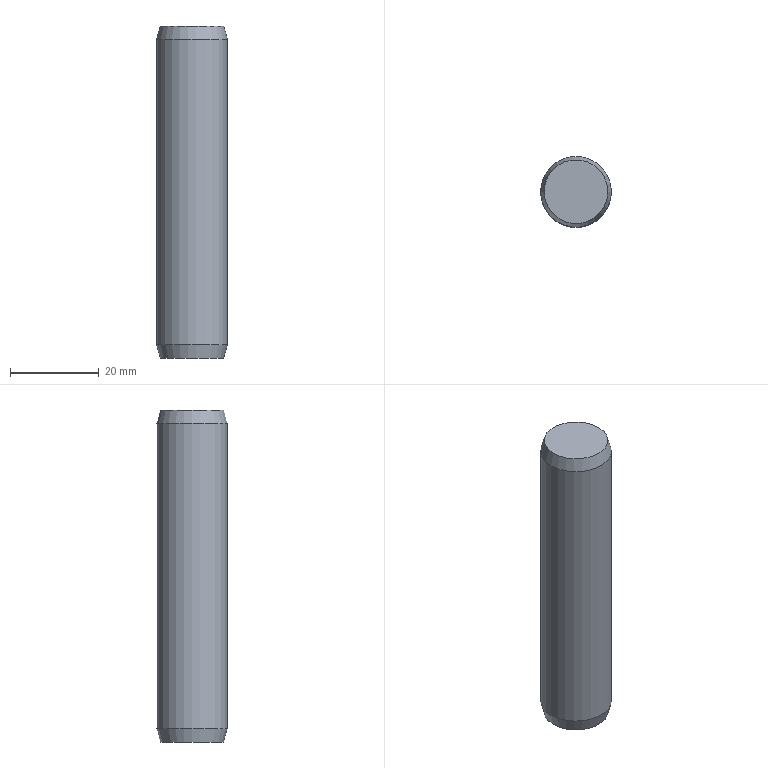Component | NX | GB-T119_1-2000_16X75 | 1 solid | 5 faces | box 16 x 16 x 75 mm | volume 14962 mm3 | plane 2 | cone 2 | cylinder 1 | commonest cylinder face diameters 16 x1
STEP:
#1=CARTESIAN_POINT('',(0.,0.,0.));
#2=DIRECTION('',(0.,0.,1.));
#3=DIRECTION('',(1.,0.,0.));
#4=AXIS2_PLACEMENT_3D('',#1,#2,#3);
#5=CARTESIAN_POINT('',(90.804,50.,10.));
#6=VERTEX_POINT('',#5);
#7=CARTESIAN_POINT('',(98.,50.,10.));
#8=DIRECTION('',(0.,0.,-1.));
#9=DIRECTION('',(-1.,0.,0.));
#10=AXIS2_PLACEMENT_3D('',#7,#8,#9);
#11=CIRCLE('',#10,7.196);
#12=CARTESIAN_POINT('',(98.,50.,10.));
#13=DIRECTION('',(0.,0.,-1.));
#14=DIRECTION('',(-1.,0.,0.));
#15=AXIS2_PLACEMENT_3D('',#12,#13,#14);
#16=PLANE('',#15);
#17=CARTESIAN_POINT('',(0.,0.));
#18=DIRECTION('',(1.,0.));
#19=AXIS2_PLACEMENT_2D('',#17,#18);
#20=CIRCLE('',#19,7.196);
#21=(GEOMETRIC_REPRESENTATION_CONTEXT(2)PARAMETRIC_REPRESENTATION_CONTEXT()REPRESENTATION_CONTEXT('',''));
#22=DEFINITIONAL_REPRESENTATION('',(#20),#21);
#23=PCURVE('',#16,#22);
#24=CARTESIAN_POINT('',(98.,50.,10.));
#25=DIRECTION('',(0.,0.,1.));
#26=DIRECTION('',(1.,0.,0.));
#27=AXIS2_PLACEMENT_3D('',#24,#25,#26);
#28=CONICAL_SURFACE('',#27,7.196,0.2618);
#29=CARTESIAN_POINT('',(9.425,-0.));
#30=DIRECTION('',(-1.,0.));
#31=VECTOR('',#30,1.);
#32=LINE('',#29,#31);
#33=(GEOMETRIC_REPRESENTATION_CONTEXT(2)PARAMETRIC_REPRESENTATION_CONTEXT()REPRESENTATION_CONTEXT('',''));
#34=DEFINITIONAL_REPRESENTATION('',(#32),#33);
#35=PCURVE('',#28,#34);
#36=SURFACE_CURVE('',#11,(#23,#35),.PCURVE_S1.);
#37=EDGE_CURVE('',#6,#6,#36,.T.);
#38=ORIENTED_EDGE('',*,*,#37,.T.);
#39=EDGE_LOOP('',(#38));
#40=FACE_BOUND('',#39,.T.);
#41=ADVANCED_FACE('',(#40),#16,.T.);
#42=CARTESIAN_POINT('',(90.,50.,13.));
#43=VERTEX_POINT('',#42);
#44=CARTESIAN_POINT('',(98.,50.,13.));
#45=DIRECTION('',(0.,0.,-1.));
#46=DIRECTION('',(-1.,0.,0.));
#47=AXIS2_PLACEMENT_3D('',#44,#45,#46);
#48=CIRCLE('',#47,8.);
#49=CARTESIAN_POINT('',(9.425,3.));
#50=DIRECTION('',(-1.,0.));
#51=VECTOR('',#50,1.);
#52=LINE('',#49,#51);
#53=(GEOMETRIC_REPRESENTATION_CONTEXT(2)PARAMETRIC_REPRESENTATION_CONTEXT()REPRESENTATION_CONTEXT('',''));
#54=DEFINITIONAL_REPRESENTATION('',(#52),#53);
#55=PCURVE('',#28,#54);
#56=CARTESIAN_POINT('',(98.,50.,85.));
#57=DIRECTION('',(0.,0.,-1.));
#58=DIRECTION('',(-1.,0.,0.));
#59=AXIS2_PLACEMENT_3D('',#56,#57,#58);
#60=CYLINDRICAL_SURFACE('',#59,8.);
#61=CARTESIAN_POINT('',(0.,72.));
#62=DIRECTION('',(1.,0.));
#63=VECTOR('',#62,1.);
#64=LINE('',#61,#63);
#65=(GEOMETRIC_REPRESENTATION_CONTEXT(2)PARAMETRIC_REPRESENTATION_CONTEXT()REPRESENTATION_CONTEXT('',''));
#66=DEFINITIONAL_REPRESENTATION('',(#64),#65);
#67=PCURVE('',#60,#66);
#68=SURFACE_CURVE('',#48,(#55,#67),.PCURVE_S1.);
#69=EDGE_CURVE('',#43,#43,#68,.T.);
#70=ORIENTED_EDGE('',*,*,#69,.T.);
#71=CARTESIAN_POINT('',(90.804,50.,10.));
#72=CARTESIAN_POINT('',(90.,50.,13.));
#73=B_SPLINE_CURVE_WITH_KNOTS('',1,(#71,#72),.UNSPECIFIED.,.F.,.F.,(2,2),(-0.,3.106),.PIECEWISE_BEZIER_KNOTS.);
#74=CARTESIAN_POINT('',(3.142,0.));
#75=DIRECTION('',(0.,1.));
#76=VECTOR('',#75,1.);
#77=LINE('',#74,#76);
#78=(GEOMETRIC_REPRESENTATION_CONTEXT(2)PARAMETRIC_REPRESENTATION_CONTEXT()REPRESENTATION_CONTEXT('',''));
#79=DEFINITIONAL_REPRESENTATION('',(#77),#78);
#80=PCURVE('',#28,#79);
#81=CARTESIAN_POINT('',(9.425,0.));
#82=DIRECTION('',(0.,1.));
#83=VECTOR('',#82,1.);
#84=LINE('',#81,#83);
#85=(GEOMETRIC_REPRESENTATION_CONTEXT(2)PARAMETRIC_REPRESENTATION_CONTEXT()REPRESENTATION_CONTEXT('',''));
#86=DEFINITIONAL_REPRESENTATION('',(#84),#85);
#87=PCURVE('',#28,#86);
#88=SEAM_CURVE('',#73,(#80,#87),.PCURVE_S1.);
#89=EDGE_CURVE('',#6,#43,#88,.T.);
#90=ORIENTED_EDGE('',*,*,#89,.F.);
#91=ORIENTED_EDGE('',*,*,#37,.F.);
#92=ORIENTED_EDGE('',*,*,#89,.T.);
#93=EDGE_LOOP('',(#70,#90,#91,#92));
#94=FACE_BOUND('',#93,.T.);
#95=ADVANCED_FACE('',(#94),#28,.T.);
#96=CARTESIAN_POINT('',(90.,50.,82.));
#97=VERTEX_POINT('',#96);
#98=CARTESIAN_POINT('',(98.,50.,82.));
#99=DIRECTION('',(0.,0.,-1.));
#100=DIRECTION('',(-1.,0.,0.));
#101=AXIS2_PLACEMENT_3D('',#98,#99,#100);
#102=CIRCLE('',#101,8.);
#103=CARTESIAN_POINT('',(0.,3.));
#104=DIRECTION('',(1.,0.));
#105=VECTOR('',#104,1.);
#106=LINE('',#103,#105);
#107=(GEOMETRIC_REPRESENTATION_CONTEXT(2)PARAMETRIC_REPRESENTATION_CONTEXT()REPRESENTATION_CONTEXT('',''));
#108=DEFINITIONAL_REPRESENTATION('',(#106),#107);
#109=PCURVE('',#60,#108);
#110=CARTESIAN_POINT('',(98.,50.,82.));
#111=DIRECTION('',(0.,0.,-1.));
#112=DIRECTION('',(-1.,0.,0.));
#113=AXIS2_PLACEMENT_3D('',#110,#111,#112);
#114=CONICAL_SURFACE('',#113,8.,0.2618);
#115=CARTESIAN_POINT('',(0.,-0.));
#116=DIRECTION('',(1.,0.));
#117=VECTOR('',#116,1.);
#118=LINE('',#115,#117);
#119=(GEOMETRIC_REPRESENTATION_CONTEXT(2)PARAMETRIC_REPRESENTATION_CONTEXT()REPRESENTATION_CONTEXT('',''));
#120=DEFINITIONAL_REPRESENTATION('',(#118),#119);
#121=PCURVE('',#114,#120);
#122=SURFACE_CURVE('',#102,(#109,#121),.PCURVE_S1.);
#123=EDGE_CURVE('',#97,#97,#122,.T.);
#124=ORIENTED_EDGE('',*,*,#123,.T.);
#125=CARTESIAN_POINT('',(90.,50.,82.));
#126=CARTESIAN_POINT('',(90.,50.,13.));
#127=B_SPLINE_CURVE_WITH_KNOTS('',1,(#125,#126),.UNSPECIFIED.,.F.,.F.,(2,2),(3.,72.),.PIECEWISE_BEZIER_KNOTS.);
#128=CARTESIAN_POINT('',(6.283,0.));
#129=DIRECTION('',(0.,1.));
#130=VECTOR('',#129,1.);
#131=LINE('',#128,#130);
#132=(GEOMETRIC_REPRESENTATION_CONTEXT(2)PARAMETRIC_REPRESENTATION_CONTEXT()REPRESENTATION_CONTEXT('',''));
#133=DEFINITIONAL_REPRESENTATION('',(#131),#132);
#134=PCURVE('',#60,#133);
#135=CARTESIAN_POINT('',(0.,0.));
#136=DIRECTION('',(0.,1.));
#137=VECTOR('',#136,1.);
#138=LINE('',#135,#137);
#139=(GEOMETRIC_REPRESENTATION_CONTEXT(2)PARAMETRIC_REPRESENTATION_CONTEXT()REPRESENTATION_CONTEXT('',''));
#140=DEFINITIONAL_REPRESENTATION('',(#138),#139);
#141=PCURVE('',#60,#140);
#142=SEAM_CURVE('',#127,(#134,#141),.PCURVE_S1.);
#143=EDGE_CURVE('',#97,#43,#142,.T.);
#144=ORIENTED_EDGE('',*,*,#143,.T.);
#145=ORIENTED_EDGE('',*,*,#69,.F.);
#146=ORIENTED_EDGE('',*,*,#143,.F.);
#147=EDGE_LOOP('',(#124,#144,#145,#146));
#148=FACE_BOUND('',#147,.T.);
#149=ADVANCED_FACE('',(#148),#60,.T.);
#150=CARTESIAN_POINT('',(90.804,50.,85.));
#151=VERTEX_POINT('',#150);
#152=CARTESIAN_POINT('',(98.,50.,85.));
#153=DIRECTION('',(0.,0.,-1.));
#154=DIRECTION('',(-1.,0.,0.));
#155=AXIS2_PLACEMENT_3D('',#152,#153,#154);
#156=CIRCLE('',#155,7.196);
#157=CARTESIAN_POINT('',(0.,-3.));
#158=DIRECTION('',(1.,0.));
#159=VECTOR('',#158,1.);
#160=LINE('',#157,#159);
#161=(GEOMETRIC_REPRESENTATION_CONTEXT(2)PARAMETRIC_REPRESENTATION_CONTEXT()REPRESENTATION_CONTEXT('',''));
#162=DEFINITIONAL_REPRESENTATION('',(#160),#161);
#163=PCURVE('',#114,#162);
#164=CARTESIAN_POINT('',(105.196,50.,85.));
#165=DIRECTION('',(0.,0.,1.));
#166=DIRECTION('',(1.,0.,0.));
#167=AXIS2_PLACEMENT_3D('',#164,#165,#166);
#168=PLANE('',#167);
#169=CARTESIAN_POINT('',(-14.392,0.));
#170=CARTESIAN_POINT('',(-14.392,12.464));
#171=CARTESIAN_POINT('',(-3.598,6.232));
#172=CARTESIAN_POINT('',(7.196,0.));
#173=CARTESIAN_POINT('',(-3.598,-6.232));
#174=CARTESIAN_POINT('',(-14.392,-12.464));
#175=CARTESIAN_POINT('',(-14.392,0.));
#176=(BOUNDED_CURVE()B_SPLINE_CURVE(2,(#169,#170,#171,#172,#173,#174,#175),.UNSPECIFIED.,.T.,.F.)B_SPLINE_CURVE_WITH_KNOTS((1,2,2,2,2,1),(-2.094,0.,2.094,4.189,6.283,8.378),.UNSPECIFIED.)CURVE()GEOMETRIC_REPRESENTATION_ITEM()RATIONAL_B_SPLINE_CURVE((1.,0.5,1.,0.5,1.,0.5,1.))REPRESENTATION_ITEM(''));
#177=(GEOMETRIC_REPRESENTATION_CONTEXT(2)PARAMETRIC_REPRESENTATION_CONTEXT()REPRESENTATION_CONTEXT('',''));
#178=DEFINITIONAL_REPRESENTATION('',(#176),#177);
#179=PCURVE('',#168,#178);
#180=SURFACE_CURVE('',#156,(#163,#179),.PCURVE_S1.);
#181=EDGE_CURVE('',#151,#151,#180,.T.);
#182=ORIENTED_EDGE('',*,*,#181,.T.);
#183=CARTESIAN_POINT('',(90.804,50.,85.));
#184=CARTESIAN_POINT('',(90.,50.,82.));
#185=B_SPLINE_CURVE_WITH_KNOTS('',1,(#183,#184),.UNSPECIFIED.,.F.,.F.,(2,2),(-3.106,-0.),.PIECEWISE_BEZIER_KNOTS.);
#186=CARTESIAN_POINT('',(6.283,0.));
#187=DIRECTION('',(0.,1.));
#188=VECTOR('',#187,1.);
#189=LINE('',#186,#188);
#190=(GEOMETRIC_REPRESENTATION_CONTEXT(2)PARAMETRIC_REPRESENTATION_CONTEXT()REPRESENTATION_CONTEXT('',''));
#191=DEFINITIONAL_REPRESENTATION('',(#189),#190);
#192=PCURVE('',#114,#191);
#193=CARTESIAN_POINT('',(0.,0.));
#194=DIRECTION('',(0.,1.));
#195=VECTOR('',#194,1.);
#196=LINE('',#193,#195);
#197=(GEOMETRIC_REPRESENTATION_CONTEXT(2)PARAMETRIC_REPRESENTATION_CONTEXT()REPRESENTATION_CONTEXT('',''));
#198=DEFINITIONAL_REPRESENTATION('',(#196),#197);
#199=PCURVE('',#114,#198);
#200=SEAM_CURVE('',#185,(#192,#199),.PCURVE_S1.);
#201=EDGE_CURVE('',#151,#97,#200,.T.);
#202=ORIENTED_EDGE('',*,*,#201,.T.);
#203=ORIENTED_EDGE('',*,*,#123,.F.);
#204=ORIENTED_EDGE('',*,*,#201,.F.);
#205=EDGE_LOOP('',(#182,#202,#203,#204));
#206=FACE_BOUND('',#205,.T.);
#207=ADVANCED_FACE('',(#206),#114,.T.);
#208=ORIENTED_EDGE('',*,*,#181,.F.);
#209=EDGE_LOOP('',(#208));
#210=FACE_BOUND('',#209,.T.);
#211=ADVANCED_FACE('',(#210),#168,.T.);
#212=CLOSED_SHELL('',(#41,#95,#149,#207,#211));
#213=MANIFOLD_SOLID_BREP('',#212);
#214=(LENGTH_UNIT()NAMED_UNIT(*)SI_UNIT(.MILLI.,.METRE.));
#215=UNCERTAINTY_MEASURE_WITH_UNIT(LENGTH_MEASURE(0.00001),#214,'','');
#216=(NAMED_UNIT(*)PLANE_ANGLE_UNIT()SI_UNIT($,.RADIAN.));
#217=(NAMED_UNIT(*)SI_UNIT($,.STERADIAN.)SOLID_ANGLE_UNIT());
#218=(GEOMETRIC_REPRESENTATION_CONTEXT(3)GLOBAL_UNCERTAINTY_ASSIGNED_CONTEXT((#215))GLOBAL_UNIT_ASSIGNED_CONTEXT((#214,#216,#217))REPRESENTATION_CONTEXT('',''));
#219=ADVANCED_BREP_SHAPE_REPRESENTATION('',(#4,#213),#218);